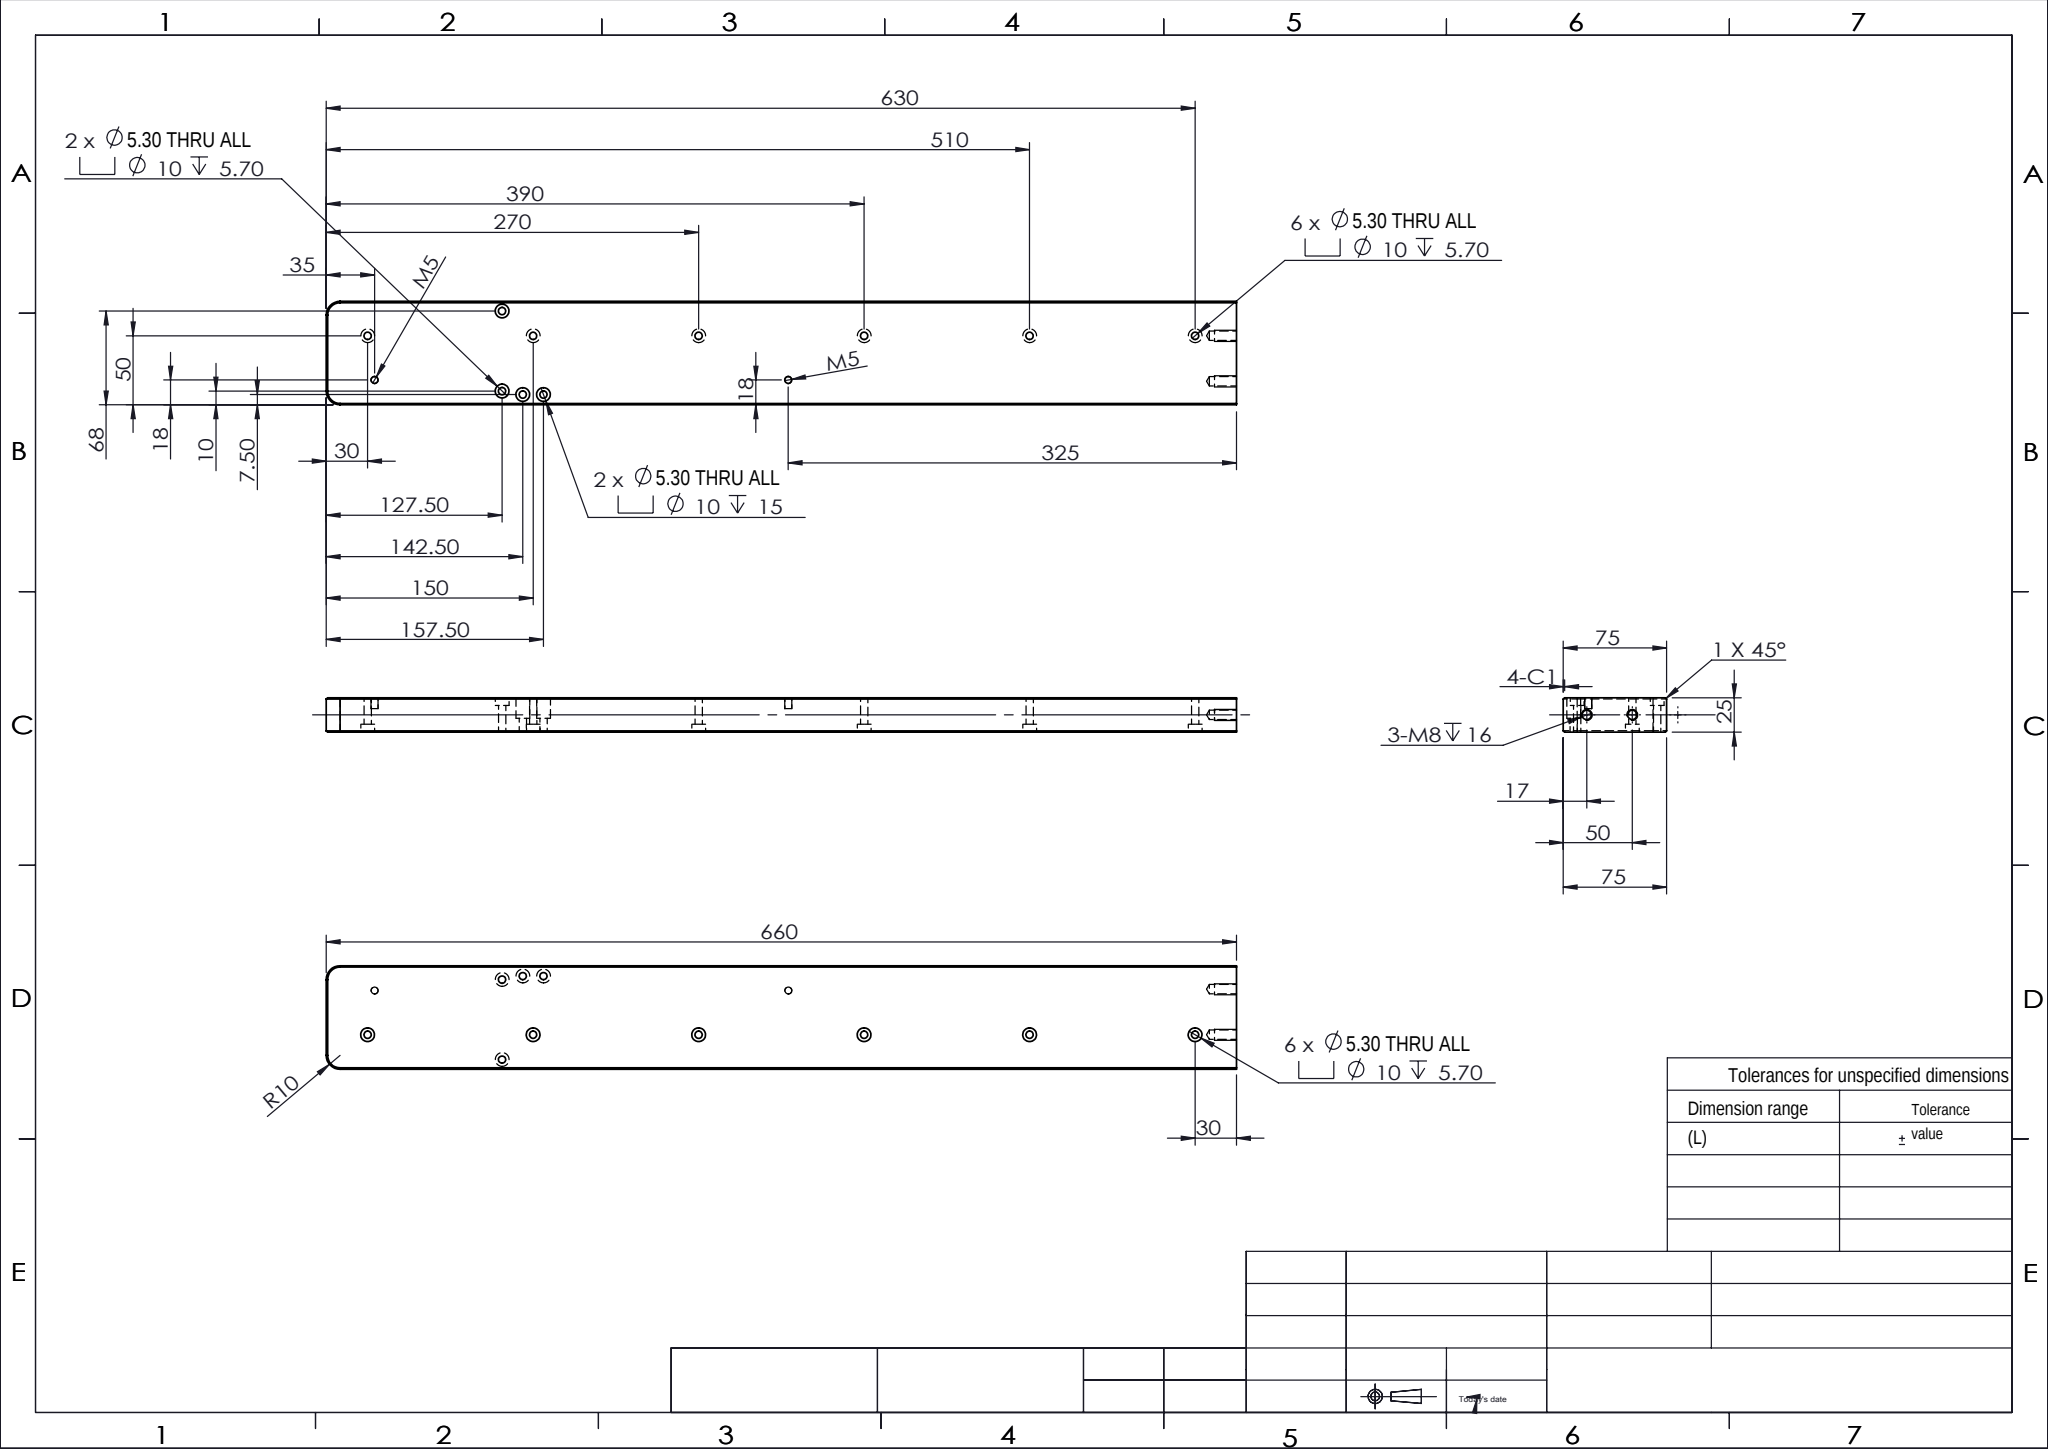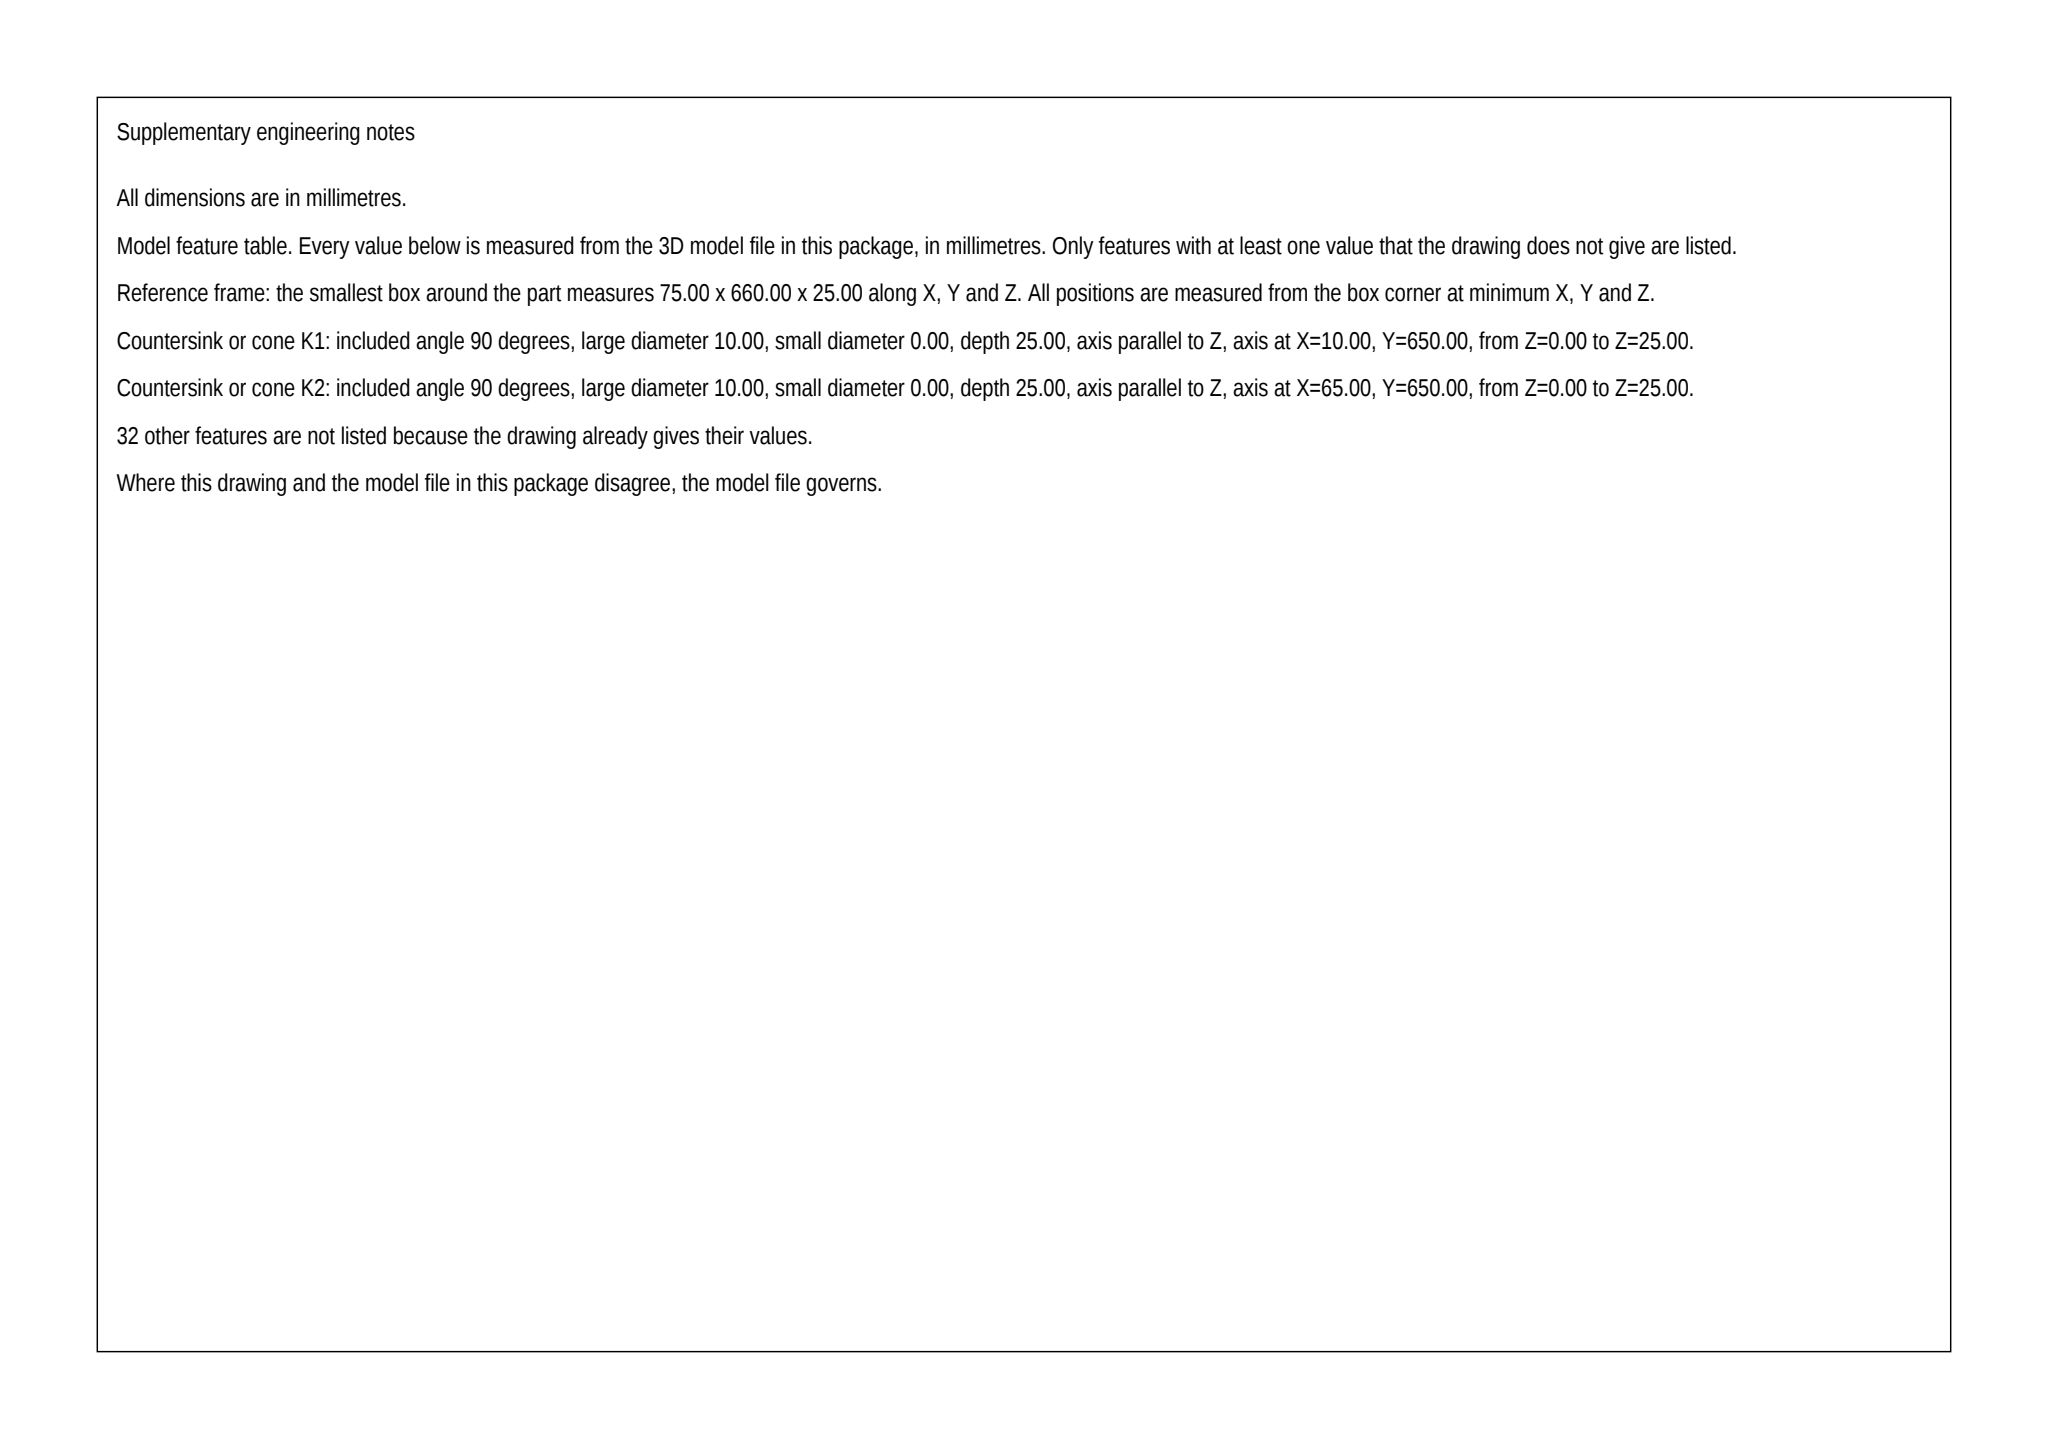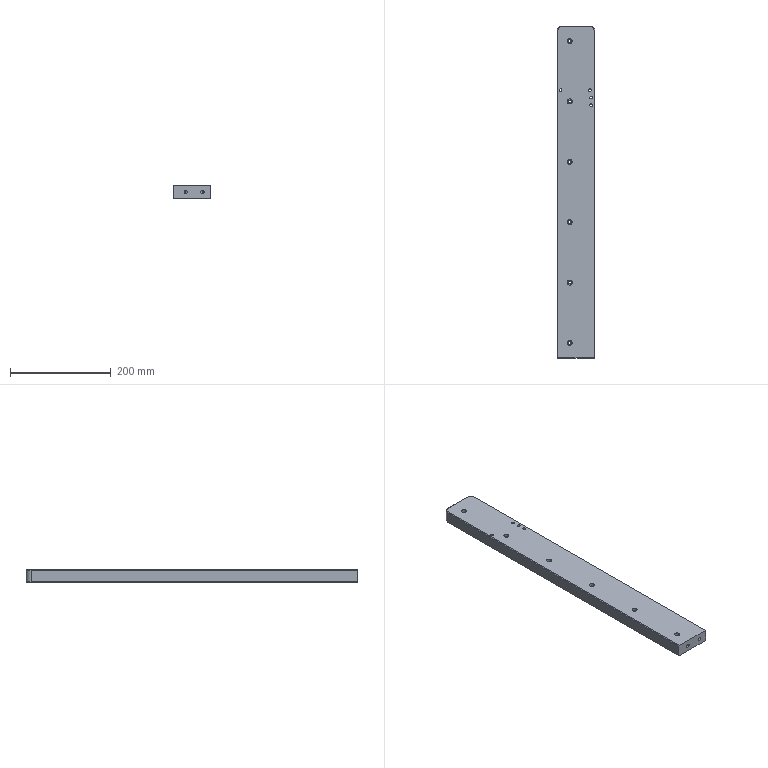Part | SolidWorks | mm | 1 solid | 82 faces | box 75 x 660 x 25 mm | volume 1223458 mm3 | cylinder 50 | plane 24 | cone 8 | commonest cylinder face diameters 5.3 x20 10 x20 5 x4 6.8 x4 20 x2
Drawing notes:
STOCK 660 X 75 X 25 | from the solid: bbox_xyz 75 x 660 x 25
8X Ø5.30 THRU, CBORE Ø10 DP 5.70 | from the solid: Ø5.3 L19.3 + coaxial Ø10 L5.7 at x25/y30,150,270,390,510,630 and x7 & x65 /y532.5
2X Ø5.30 THRU, CBORE Ø10 DP 15, CL 7.50 FROM TOP EDGE | from the solid: Ø5.3 L10 + coaxial Ø10 L15 at x67.5 (75-67.5=7.5), y502.5 & 517.5
2X M5 DP 8, CL 18 FROM TOP EDGE | from the solid: Ø5.0 z-axis L8 at [57,325] and [57,625]; 75-57=18
4X M8 DP 16, 2 EA END FACE, CL 17 & 50 FROM TOP EDGE, 12.50 FROM EA FACE | from the solid: Ø6.8 y-axis L19.75 (118° pt) at x58 (75-58=17) & x25 (75-25=50), z=12.5 of 25 thk, on y=0 and y=660